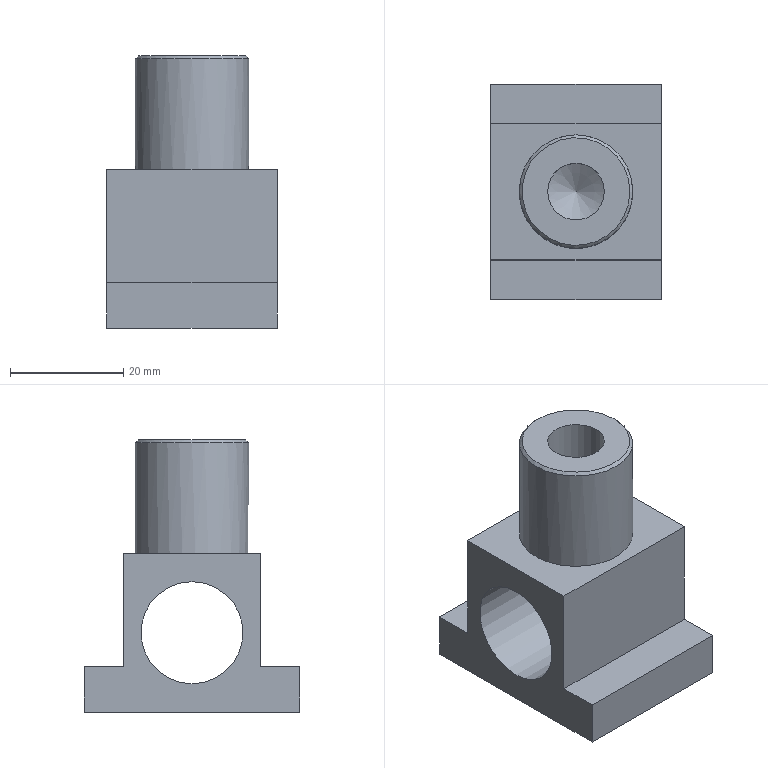Component | NX | 5 | 1 solid | 16 faces | box 30 x 38 x 48 mm | volume 20512 mm3 | plane 11 | cylinder 3 | cone 2 | commonest cylinder face diameters 18 x1 20 x1 10 x1
STEP:
#1=CARTESIAN_POINT('',(0.,0.,0.));
#2=DIRECTION('',(0.,0.,1.));
#3=DIRECTION('',(1.,0.,0.));
#4=AXIS2_PLACEMENT_3D('',#1,#2,#3);
#5=CARTESIAN_POINT('',(49.,-19.,9.));
#6=VERTEX_POINT('',#5);
#7=CARTESIAN_POINT('',(49.,-19.,1.));
#8=VERTEX_POINT('',#7);
#9=CARTESIAN_POINT('',(49.,-19.,9.));
#10=DIRECTION('',(0.,0.,-1.));
#11=VECTOR('',#10,1.);
#12=LINE('',#9,#11);
#13=CARTESIAN_POINT('',(79.,-19.,9.));
#14=DIRECTION('',(0.,1.,0.));
#15=DIRECTION('',(0.,0.,1.));
#16=AXIS2_PLACEMENT_3D('',#13,#14,#15);
#17=PLANE('',#16);
#18=CARTESIAN_POINT('',(0.,-30.));
#19=DIRECTION('',(-1.,0.));
#20=VECTOR('',#19,1.);
#21=LINE('',#18,#20);
#22=(GEOMETRIC_REPRESENTATION_CONTEXT(2)PARAMETRIC_REPRESENTATION_CONTEXT()REPRESENTATION_CONTEXT('',''));
#23=DEFINITIONAL_REPRESENTATION('',(#21),#22);
#24=PCURVE('',#17,#23);
#25=CARTESIAN_POINT('',(49.,-0.,1.));
#26=DIRECTION('',(1.,0.,0.));
#27=DIRECTION('',(0.,0.,-1.));
#28=AXIS2_PLACEMENT_3D('',#25,#26,#27);
#29=PLANE('',#28);
#30=CARTESIAN_POINT('',(-8.,-19.));
#31=DIRECTION('',(1.,0.));
#32=VECTOR('',#31,1.);
#33=LINE('',#30,#32);
#34=(GEOMETRIC_REPRESENTATION_CONTEXT(2)PARAMETRIC_REPRESENTATION_CONTEXT()REPRESENTATION_CONTEXT('',''));
#35=DEFINITIONAL_REPRESENTATION('',(#33),#34);
#36=PCURVE('',#29,#35);
#37=SURFACE_CURVE('',#12,(#24,#36),.PCURVE_S1.);
#38=EDGE_CURVE('',#6,#8,#37,.T.);
#39=ORIENTED_EDGE('',*,*,#38,.T.);
#40=CARTESIAN_POINT('',(79.,-19.,1.));
#41=VERTEX_POINT('',#40);
#42=CARTESIAN_POINT('',(79.,-19.,1.));
#43=DIRECTION('',(-1.,0.,0.));
#44=VECTOR('',#43,1.);
#45=LINE('',#42,#44);
#46=CARTESIAN_POINT('',(-8.,0.));
#47=DIRECTION('',(0.,-1.));
#48=VECTOR('',#47,1.);
#49=LINE('',#46,#48);
#50=(GEOMETRIC_REPRESENTATION_CONTEXT(2)PARAMETRIC_REPRESENTATION_CONTEXT()REPRESENTATION_CONTEXT('',''));
#51=DEFINITIONAL_REPRESENTATION('',(#49),#50);
#52=PCURVE('',#17,#51);
#53=CARTESIAN_POINT('',(79.,-19.,1.));
#54=DIRECTION('',(0.,-0.,1.));
#55=DIRECTION('',(0.,-1.,-0.));
#56=AXIS2_PLACEMENT_3D('',#53,#54,#55);
#57=PLANE('',#56);
#58=CARTESIAN_POINT('',(0.,0.));
#59=DIRECTION('',(0.,-1.));
#60=VECTOR('',#59,1.);
#61=LINE('',#58,#60);
#62=(GEOMETRIC_REPRESENTATION_CONTEXT(2)PARAMETRIC_REPRESENTATION_CONTEXT()REPRESENTATION_CONTEXT('',''));
#63=DEFINITIONAL_REPRESENTATION('',(#61),#62);
#64=PCURVE('',#57,#63);
#65=SURFACE_CURVE('',#45,(#52,#64),.PCURVE_S1.);
#66=EDGE_CURVE('',#41,#8,#65,.T.);
#67=ORIENTED_EDGE('',*,*,#66,.F.);
#68=CARTESIAN_POINT('',(79.,-19.,9.));
#69=VERTEX_POINT('',#68);
#70=CARTESIAN_POINT('',(79.,-19.,9.));
#71=DIRECTION('',(0.,0.,-1.));
#72=VECTOR('',#71,1.);
#73=LINE('',#70,#72);
#74=CARTESIAN_POINT('',(0.,0.));
#75=DIRECTION('',(-1.,0.));
#76=VECTOR('',#75,1.);
#77=LINE('',#74,#76);
#78=(GEOMETRIC_REPRESENTATION_CONTEXT(2)PARAMETRIC_REPRESENTATION_CONTEXT()REPRESENTATION_CONTEXT('',''));
#79=DEFINITIONAL_REPRESENTATION('',(#77),#78);
#80=PCURVE('',#17,#79);
#81=CARTESIAN_POINT('',(79.,-0.,1.));
#82=DIRECTION('',(1.,0.,0.));
#83=DIRECTION('',(0.,0.,-1.));
#84=AXIS2_PLACEMENT_3D('',#81,#82,#83);
#85=PLANE('',#84);
#86=CARTESIAN_POINT('',(-8.,-19.));
#87=DIRECTION('',(1.,0.));
#88=VECTOR('',#87,1.);
#89=LINE('',#86,#88);
#90=(GEOMETRIC_REPRESENTATION_CONTEXT(2)PARAMETRIC_REPRESENTATION_CONTEXT()REPRESENTATION_CONTEXT('',''));
#91=DEFINITIONAL_REPRESENTATION('',(#89),#90);
#92=PCURVE('',#85,#91);
#93=SURFACE_CURVE('',#73,(#80,#92),.PCURVE_S1.);
#94=EDGE_CURVE('',#69,#41,#93,.T.);
#95=ORIENTED_EDGE('',*,*,#94,.F.);
#96=CARTESIAN_POINT('',(79.,-19.,9.));
#97=DIRECTION('',(-1.,0.,0.));
#98=VECTOR('',#97,1.);
#99=LINE('',#96,#98);
#100=CARTESIAN_POINT('',(0.,0.));
#101=DIRECTION('',(0.,-1.));
#102=VECTOR('',#101,1.);
#103=LINE('',#100,#102);
#104=(GEOMETRIC_REPRESENTATION_CONTEXT(2)PARAMETRIC_REPRESENTATION_CONTEXT()REPRESENTATION_CONTEXT('',''));
#105=DEFINITIONAL_REPRESENTATION('',(#103),#104);
#106=PCURVE('',#17,#105);
#107=CARTESIAN_POINT('',(79.,-12.,9.));
#108=DIRECTION('',(0.,0.,-1.));
#109=DIRECTION('',(-1.,0.,0.));
#110=AXIS2_PLACEMENT_3D('',#107,#108,#109);
#111=PLANE('',#110);
#112=CARTESIAN_POINT('',(0.,-7.));
#113=DIRECTION('',(1.,0.));
#114=VECTOR('',#113,1.);
#115=LINE('',#112,#114);
#116=(GEOMETRIC_REPRESENTATION_CONTEXT(2)PARAMETRIC_REPRESENTATION_CONTEXT()REPRESENTATION_CONTEXT('',''));
#117=DEFINITIONAL_REPRESENTATION('',(#115),#116);
#118=PCURVE('',#111,#117);
#119=SURFACE_CURVE('',#99,(#106,#118),.PCURVE_S1.);
#120=EDGE_CURVE('',#69,#6,#119,.T.);
#121=ORIENTED_EDGE('',*,*,#120,.T.);
#122=EDGE_LOOP('',(#39,#67,#95,#121));
#123=FACE_BOUND('',#122,.T.);
#124=ADVANCED_FACE('',(#123),#17,.F.);
#125=CARTESIAN_POINT('',(49.,19.,1.));
#126=VERTEX_POINT('',#125);
#127=CARTESIAN_POINT('',(49.,-19.,1.));
#128=DIRECTION('',(0.,1.,0.));
#129=VECTOR('',#128,1.);
#130=LINE('',#127,#129);
#131=CARTESIAN_POINT('',(0.,-30.));
#132=DIRECTION('',(-1.,0.));
#133=VECTOR('',#132,1.);
#134=LINE('',#131,#133);
#135=(GEOMETRIC_REPRESENTATION_CONTEXT(2)PARAMETRIC_REPRESENTATION_CONTEXT()REPRESENTATION_CONTEXT('',''));
#136=DEFINITIONAL_REPRESENTATION('',(#134),#135);
#137=PCURVE('',#57,#136);
#138=CARTESIAN_POINT('',(0.,-19.));
#139=DIRECTION('',(-0.,1.));
#140=VECTOR('',#139,1.);
#141=LINE('',#138,#140);
#142=(GEOMETRIC_REPRESENTATION_CONTEXT(2)PARAMETRIC_REPRESENTATION_CONTEXT()REPRESENTATION_CONTEXT('',''));
#143=DEFINITIONAL_REPRESENTATION('',(#141),#142);
#144=PCURVE('',#29,#143);
#145=SURFACE_CURVE('',#130,(#137,#144),.PCURVE_S1.);
#146=EDGE_CURVE('',#8,#126,#145,.T.);
#147=ORIENTED_EDGE('',*,*,#146,.T.);
#148=CARTESIAN_POINT('',(79.,19.,1.));
#149=VERTEX_POINT('',#148);
#150=CARTESIAN_POINT('',(79.,19.,1.));
#151=DIRECTION('',(-1.,0.,0.));
#152=VECTOR('',#151,1.);
#153=LINE('',#150,#152);
#154=CARTESIAN_POINT('',(-38.,0.));
#155=DIRECTION('',(0.,-1.));
#156=VECTOR('',#155,1.);
#157=LINE('',#154,#156);
#158=(GEOMETRIC_REPRESENTATION_CONTEXT(2)PARAMETRIC_REPRESENTATION_CONTEXT()REPRESENTATION_CONTEXT('',''));
#159=DEFINITIONAL_REPRESENTATION('',(#157),#158);
#160=PCURVE('',#57,#159);
#161=CARTESIAN_POINT('',(79.,19.,1.));
#162=DIRECTION('',(0.,-1.,0.));
#163=DIRECTION('',(0.,0.,-1.));
#164=AXIS2_PLACEMENT_3D('',#161,#162,#163);
#165=PLANE('',#164);
#166=CARTESIAN_POINT('',(0.,0.));
#167=DIRECTION('',(0.,-1.));
#168=VECTOR('',#167,1.);
#169=LINE('',#166,#168);
#170=(GEOMETRIC_REPRESENTATION_CONTEXT(2)PARAMETRIC_REPRESENTATION_CONTEXT()REPRESENTATION_CONTEXT('',''));
#171=DEFINITIONAL_REPRESENTATION('',(#169),#170);
#172=PCURVE('',#165,#171);
#173=SURFACE_CURVE('',#153,(#160,#172),.PCURVE_S1.);
#174=EDGE_CURVE('',#149,#126,#173,.T.);
#175=ORIENTED_EDGE('',*,*,#174,.F.);
#176=CARTESIAN_POINT('',(79.,-19.,1.));
#177=DIRECTION('',(0.,1.,0.));
#178=VECTOR('',#177,1.);
#179=LINE('',#176,#178);
#180=CARTESIAN_POINT('',(0.,0.));
#181=DIRECTION('',(-1.,0.));
#182=VECTOR('',#181,1.);
#183=LINE('',#180,#182);
#184=(GEOMETRIC_REPRESENTATION_CONTEXT(2)PARAMETRIC_REPRESENTATION_CONTEXT()REPRESENTATION_CONTEXT('',''));
#185=DEFINITIONAL_REPRESENTATION('',(#183),#184);
#186=PCURVE('',#57,#185);
#187=CARTESIAN_POINT('',(0.,-19.));
#188=DIRECTION('',(-0.,1.));
#189=VECTOR('',#188,1.);
#190=LINE('',#187,#189);
#191=(GEOMETRIC_REPRESENTATION_CONTEXT(2)PARAMETRIC_REPRESENTATION_CONTEXT()REPRESENTATION_CONTEXT('',''));
#192=DEFINITIONAL_REPRESENTATION('',(#190),#191);
#193=PCURVE('',#85,#192);
#194=SURFACE_CURVE('',#179,(#186,#193),.PCURVE_S1.);
#195=EDGE_CURVE('',#41,#149,#194,.T.);
#196=ORIENTED_EDGE('',*,*,#195,.F.);
#197=ORIENTED_EDGE('',*,*,#66,.T.);
#198=EDGE_LOOP('',(#147,#175,#196,#197));
#199=FACE_BOUND('',#198,.T.);
#200=ADVANCED_FACE('',(#199),#57,.F.);
#201=CARTESIAN_POINT('',(49.,19.,9.));
#202=VERTEX_POINT('',#201);
#203=CARTESIAN_POINT('',(49.,19.,1.));
#204=DIRECTION('',(0.,0.,1.));
#205=VECTOR('',#204,1.);
#206=LINE('',#203,#205);
#207=CARTESIAN_POINT('',(0.,-30.));
#208=DIRECTION('',(-1.,0.));
#209=VECTOR('',#208,1.);
#210=LINE('',#207,#209);
#211=(GEOMETRIC_REPRESENTATION_CONTEXT(2)PARAMETRIC_REPRESENTATION_CONTEXT()REPRESENTATION_CONTEXT('',''));
#212=DEFINITIONAL_REPRESENTATION('',(#210),#211);
#213=PCURVE('',#165,#212);
#214=CARTESIAN_POINT('',(0.,19.));
#215=DIRECTION('',(-1.,0.));
#216=VECTOR('',#215,1.);
#217=LINE('',#214,#216);
#218=(GEOMETRIC_REPRESENTATION_CONTEXT(2)PARAMETRIC_REPRESENTATION_CONTEXT()REPRESENTATION_CONTEXT('',''));
#219=DEFINITIONAL_REPRESENTATION('',(#217),#218);
#220=PCURVE('',#29,#219);
#221=SURFACE_CURVE('',#206,(#213,#220),.PCURVE_S1.);
#222=EDGE_CURVE('',#126,#202,#221,.T.);
#223=ORIENTED_EDGE('',*,*,#222,.T.);
#224=CARTESIAN_POINT('',(79.,19.,9.));
#225=VERTEX_POINT('',#224);
#226=CARTESIAN_POINT('',(79.,19.,9.));
#227=DIRECTION('',(-1.,0.,0.));
#228=VECTOR('',#227,1.);
#229=LINE('',#226,#228);
#230=CARTESIAN_POINT('',(-8.,0.));
#231=DIRECTION('',(0.,-1.));
#232=VECTOR('',#231,1.);
#233=LINE('',#230,#232);
#234=(GEOMETRIC_REPRESENTATION_CONTEXT(2)PARAMETRIC_REPRESENTATION_CONTEXT()REPRESENTATION_CONTEXT('',''));
#235=DEFINITIONAL_REPRESENTATION('',(#233),#234);
#236=PCURVE('',#165,#235);
#237=CARTESIAN_POINT('',(79.,19.,9.));
#238=DIRECTION('',(0.,0.,-1.));
#239=DIRECTION('',(0.,1.,0.));
#240=AXIS2_PLACEMENT_3D('',#237,#238,#239);
#241=PLANE('',#240);
#242=CARTESIAN_POINT('',(0.,0.));
#243=DIRECTION('',(0.,-1.));
#244=VECTOR('',#243,1.);
#245=LINE('',#242,#244);
#246=(GEOMETRIC_REPRESENTATION_CONTEXT(2)PARAMETRIC_REPRESENTATION_CONTEXT()REPRESENTATION_CONTEXT('',''));
#247=DEFINITIONAL_REPRESENTATION('',(#245),#246);
#248=PCURVE('',#241,#247);
#249=SURFACE_CURVE('',#229,(#236,#248),.PCURVE_S1.);
#250=EDGE_CURVE('',#225,#202,#249,.T.);
#251=ORIENTED_EDGE('',*,*,#250,.F.);
#252=CARTESIAN_POINT('',(79.,19.,1.));
#253=DIRECTION('',(0.,0.,1.));
#254=VECTOR('',#253,1.);
#255=LINE('',#252,#254);
#256=CARTESIAN_POINT('',(0.,0.));
#257=DIRECTION('',(-1.,0.));
#258=VECTOR('',#257,1.);
#259=LINE('',#256,#258);
#260=(GEOMETRIC_REPRESENTATION_CONTEXT(2)PARAMETRIC_REPRESENTATION_CONTEXT()REPRESENTATION_CONTEXT('',''));
#261=DEFINITIONAL_REPRESENTATION('',(#259),#260);
#262=PCURVE('',#165,#261);
#263=CARTESIAN_POINT('',(0.,19.));
#264=DIRECTION('',(-1.,0.));
#265=VECTOR('',#264,1.);
#266=LINE('',#263,#265);
#267=(GEOMETRIC_REPRESENTATION_CONTEXT(2)PARAMETRIC_REPRESENTATION_CONTEXT()REPRESENTATION_CONTEXT('',''));
#268=DEFINITIONAL_REPRESENTATION('',(#266),#267);
#269=PCURVE('',#85,#268);
#270=SURFACE_CURVE('',#255,(#262,#269),.PCURVE_S1.);
#271=EDGE_CURVE('',#149,#225,#270,.T.);
#272=ORIENTED_EDGE('',*,*,#271,.F.);
#273=ORIENTED_EDGE('',*,*,#174,.T.);
#274=EDGE_LOOP('',(#223,#251,#272,#273));
#275=FACE_BOUND('',#274,.T.);
#276=ADVANCED_FACE('',(#275),#165,.F.);
#277=CARTESIAN_POINT('',(49.,12.,9.));
#278=VERTEX_POINT('',#277);
#279=CARTESIAN_POINT('',(49.,19.,9.));
#280=DIRECTION('',(0.,-1.,-0.));
#281=VECTOR('',#280,1.);
#282=LINE('',#279,#281);
#283=CARTESIAN_POINT('',(0.,-30.));
#284=DIRECTION('',(-1.,0.));
#285=VECTOR('',#284,1.);
#286=LINE('',#283,#285);
#287=(GEOMETRIC_REPRESENTATION_CONTEXT(2)PARAMETRIC_REPRESENTATION_CONTEXT()REPRESENTATION_CONTEXT('',''));
#288=DEFINITIONAL_REPRESENTATION('',(#286),#287);
#289=PCURVE('',#241,#288);
#290=CARTESIAN_POINT('',(-8.,19.));
#291=DIRECTION('',(0.,-1.));
#292=VECTOR('',#291,1.);
#293=LINE('',#290,#292);
#294=(GEOMETRIC_REPRESENTATION_CONTEXT(2)PARAMETRIC_REPRESENTATION_CONTEXT()REPRESENTATION_CONTEXT('',''));
#295=DEFINITIONAL_REPRESENTATION('',(#293),#294);
#296=PCURVE('',#29,#295);
#297=SURFACE_CURVE('',#282,(#289,#296),.PCURVE_S1.);
#298=EDGE_CURVE('',#202,#278,#297,.T.);
#299=ORIENTED_EDGE('',*,*,#298,.T.);
#300=CARTESIAN_POINT('',(79.,12.,9.));
#301=VERTEX_POINT('',#300);
#302=CARTESIAN_POINT('',(79.,12.,9.));
#303=DIRECTION('',(-1.,0.,0.));
#304=VECTOR('',#303,1.);
#305=LINE('',#302,#304);
#306=CARTESIAN_POINT('',(-7.,0.));
#307=DIRECTION('',(0.,-1.));
#308=VECTOR('',#307,1.);
#309=LINE('',#306,#308);
#310=(GEOMETRIC_REPRESENTATION_CONTEXT(2)PARAMETRIC_REPRESENTATION_CONTEXT()REPRESENTATION_CONTEXT('',''));
#311=DEFINITIONAL_REPRESENTATION('',(#309),#310);
#312=PCURVE('',#241,#311);
#313=CARTESIAN_POINT('',(79.,12.,9.));
#314=DIRECTION('',(0.,-1.,-0.));
#315=DIRECTION('',(0.,0.,-1.));
#316=AXIS2_PLACEMENT_3D('',#313,#314,#315);
#317=PLANE('',#316);
#318=CARTESIAN_POINT('',(0.,0.));
#319=DIRECTION('',(0.,-1.));
#320=VECTOR('',#319,1.);
#321=LINE('',#318,#320);
#322=(GEOMETRIC_REPRESENTATION_CONTEXT(2)PARAMETRIC_REPRESENTATION_CONTEXT()REPRESENTATION_CONTEXT('',''));
#323=DEFINITIONAL_REPRESENTATION('',(#321),#322);
#324=PCURVE('',#317,#323);
#325=SURFACE_CURVE('',#305,(#312,#324),.PCURVE_S1.);
#326=EDGE_CURVE('',#301,#278,#325,.T.);
#327=ORIENTED_EDGE('',*,*,#326,.F.);
#328=CARTESIAN_POINT('',(79.,19.,9.));
#329=DIRECTION('',(0.,-1.,-0.));
#330=VECTOR('',#329,1.);
#331=LINE('',#328,#330);
#332=CARTESIAN_POINT('',(0.,0.));
#333=DIRECTION('',(-1.,0.));
#334=VECTOR('',#333,1.);
#335=LINE('',#332,#334);
#336=(GEOMETRIC_REPRESENTATION_CONTEXT(2)PARAMETRIC_REPRESENTATION_CONTEXT()REPRESENTATION_CONTEXT('',''));
#337=DEFINITIONAL_REPRESENTATION('',(#335),#336);
#338=PCURVE('',#241,#337);
#339=CARTESIAN_POINT('',(-8.,19.));
#340=DIRECTION('',(0.,-1.));
#341=VECTOR('',#340,1.);
#342=LINE('',#339,#341);
#343=(GEOMETRIC_REPRESENTATION_CONTEXT(2)PARAMETRIC_REPRESENTATION_CONTEXT()REPRESENTATION_CONTEXT('',''));
#344=DEFINITIONAL_REPRESENTATION('',(#342),#343);
#345=PCURVE('',#85,#344);
#346=SURFACE_CURVE('',#331,(#338,#345),.PCURVE_S1.);
#347=EDGE_CURVE('',#225,#301,#346,.T.);
#348=ORIENTED_EDGE('',*,*,#347,.F.);
#349=ORIENTED_EDGE('',*,*,#250,.T.);
#350=EDGE_LOOP('',(#299,#327,#348,#349));
#351=FACE_BOUND('',#350,.T.);
#352=ADVANCED_FACE('',(#351),#241,.F.);
#353=CARTESIAN_POINT('',(49.,12.,29.));
#354=VERTEX_POINT('',#353);
#355=CARTESIAN_POINT('',(49.,12.,9.));
#356=DIRECTION('',(0.,-0.,1.));
#357=VECTOR('',#356,1.);
#358=LINE('',#355,#357);
#359=CARTESIAN_POINT('',(0.,-30.));
#360=DIRECTION('',(-1.,0.));
#361=VECTOR('',#360,1.);
#362=LINE('',#359,#361);
#363=(GEOMETRIC_REPRESENTATION_CONTEXT(2)PARAMETRIC_REPRESENTATION_CONTEXT()REPRESENTATION_CONTEXT('',''));
#364=DEFINITIONAL_REPRESENTATION('',(#362),#363);
#365=PCURVE('',#317,#364);
#366=CARTESIAN_POINT('',(-8.,12.));
#367=DIRECTION('',(-1.,-0.));
#368=VECTOR('',#367,1.);
#369=LINE('',#366,#368);
#370=(GEOMETRIC_REPRESENTATION_CONTEXT(2)PARAMETRIC_REPRESENTATION_CONTEXT()REPRESENTATION_CONTEXT('',''));
#371=DEFINITIONAL_REPRESENTATION('',(#369),#370);
#372=PCURVE('',#29,#371);
#373=SURFACE_CURVE('',#358,(#365,#372),.PCURVE_S1.);
#374=EDGE_CURVE('',#278,#354,#373,.T.);
#375=ORIENTED_EDGE('',*,*,#374,.T.);
#376=CARTESIAN_POINT('',(79.,12.,29.));
#377=VERTEX_POINT('',#376);
#378=CARTESIAN_POINT('',(79.,12.,29.));
#379=DIRECTION('',(-1.,0.,0.));
#380=VECTOR('',#379,1.);
#381=LINE('',#378,#380);
#382=CARTESIAN_POINT('',(-20.,0.));
#383=DIRECTION('',(0.,-1.));
#384=VECTOR('',#383,1.);
#385=LINE('',#382,#384);
#386=(GEOMETRIC_REPRESENTATION_CONTEXT(2)PARAMETRIC_REPRESENTATION_CONTEXT()REPRESENTATION_CONTEXT('',''));
#387=DEFINITIONAL_REPRESENTATION('',(#385),#386);
#388=PCURVE('',#317,#387);
#389=CARTESIAN_POINT('',(79.,12.,29.));
#390=DIRECTION('',(0.,0.,-1.));
#391=DIRECTION('',(-1.,0.,0.));
#392=AXIS2_PLACEMENT_3D('',#389,#390,#391);
#393=PLANE('',#392);
#394=CARTESIAN_POINT('',(0.,0.));
#395=DIRECTION('',(1.,0.));
#396=VECTOR('',#395,1.);
#397=LINE('',#394,#396);
#398=(GEOMETRIC_REPRESENTATION_CONTEXT(2)PARAMETRIC_REPRESENTATION_CONTEXT()REPRESENTATION_CONTEXT('',''));
#399=DEFINITIONAL_REPRESENTATION('',(#397),#398);
#400=PCURVE('',#393,#399);
#401=SURFACE_CURVE('',#381,(#388,#400),.PCURVE_S1.);
#402=EDGE_CURVE('',#377,#354,#401,.T.);
#403=ORIENTED_EDGE('',*,*,#402,.F.);
#404=CARTESIAN_POINT('',(79.,12.,9.));
#405=DIRECTION('',(0.,-0.,1.));
#406=VECTOR('',#405,1.);
#407=LINE('',#404,#406);
#408=CARTESIAN_POINT('',(0.,0.));
#409=DIRECTION('',(-1.,0.));
#410=VECTOR('',#409,1.);
#411=LINE('',#408,#410);
#412=(GEOMETRIC_REPRESENTATION_CONTEXT(2)PARAMETRIC_REPRESENTATION_CONTEXT()REPRESENTATION_CONTEXT('',''));
#413=DEFINITIONAL_REPRESENTATION('',(#411),#412);
#414=PCURVE('',#317,#413);
#415=CARTESIAN_POINT('',(-8.,12.));
#416=DIRECTION('',(-1.,-0.));
#417=VECTOR('',#416,1.);
#418=LINE('',#415,#417);
#419=(GEOMETRIC_REPRESENTATION_CONTEXT(2)PARAMETRIC_REPRESENTATION_CONTEXT()REPRESENTATION_CONTEXT('',''));
#420=DEFINITIONAL_REPRESENTATION('',(#418),#419);
#421=PCURVE('',#85,#420);
#422=SURFACE_CURVE('',#407,(#414,#421),.PCURVE_S1.);
#423=EDGE_CURVE('',#301,#377,#422,.T.);
#424=ORIENTED_EDGE('',*,*,#423,.F.);
#425=ORIENTED_EDGE('',*,*,#326,.T.);
#426=EDGE_LOOP('',(#375,#403,#424,#425));
#427=FACE_BOUND('',#426,.T.);
#428=ADVANCED_FACE('',(#427),#317,.F.);
#429=CARTESIAN_POINT('',(64.,10.,29.));
#430=VERTEX_POINT('',#429);
#431=CARTESIAN_POINT('',(64.,-0.,29.));
#432=DIRECTION('',(0.,0.,1.));
#433=DIRECTION('',(0.,1.,0.));
#434=AXIS2_PLACEMENT_3D('',#431,#432,#433);
#435=CIRCLE('',#434,10.);
#436=CARTESIAN_POINT('',(15.,-2.));
#437=CARTESIAN_POINT('',(32.321,-2.));
#438=CARTESIAN_POINT('',(23.66,-17.));
#439=CARTESIAN_POINT('',(15.,-32.));
#440=CARTESIAN_POINT('',(6.34,-17.));
#441=CARTESIAN_POINT('',(-2.321,-2.));
#442=CARTESIAN_POINT('',(15.,-2.));
#443=(BOUNDED_CURVE()B_SPLINE_CURVE(2,(#436,#437,#438,#439,#440,#441,#442),.UNSPECIFIED.,.T.,.F.)B_SPLINE_CURVE_WITH_KNOTS((1,2,2,2,2,1),(-2.094,0.,2.094,4.189,6.283,8.378),.UNSPECIFIED.)CURVE()GEOMETRIC_REPRESENTATION_ITEM()RATIONAL_B_SPLINE_CURVE((1.,0.5,1.,0.5,1.,0.5,1.))REPRESENTATION_ITEM(''));
#444=(GEOMETRIC_REPRESENTATION_CONTEXT(2)PARAMETRIC_REPRESENTATION_CONTEXT()REPRESENTATION_CONTEXT('',''));
#445=DEFINITIONAL_REPRESENTATION('',(#443),#444);
#446=PCURVE('',#393,#445);
#447=CARTESIAN_POINT('',(64.,-0.,49.));
#448=DIRECTION('',(0.,0.,-1.));
#449=DIRECTION('',(-1.,0.,0.));
#450=AXIS2_PLACEMENT_3D('',#447,#448,#449);
#451=CYLINDRICAL_SURFACE('',#450,10.);
#452=CARTESIAN_POINT('',(7.854,20.));
#453=DIRECTION('',(-1.,0.));
#454=VECTOR('',#453,1.);
#455=LINE('',#452,#454);
#456=(GEOMETRIC_REPRESENTATION_CONTEXT(2)PARAMETRIC_REPRESENTATION_CONTEXT()REPRESENTATION_CONTEXT('',''));
#457=DEFINITIONAL_REPRESENTATION('',(#455),#456);
#458=PCURVE('',#451,#457);
#459=SURFACE_CURVE('',#435,(#446,#458),.PCURVE_S1.);
#460=EDGE_CURVE('',#430,#430,#459,.T.);
#461=ORIENTED_EDGE('',*,*,#460,.F.);
#462=EDGE_LOOP('',(#461));
#463=FACE_BOUND('',#462,.T.);
#464=CARTESIAN_POINT('',(49.,-12.,29.));
#465=VERTEX_POINT('',#464);
#466=CARTESIAN_POINT('',(49.,12.,29.));
#467=DIRECTION('',(0.,-1.,0.));
#468=VECTOR('',#467,1.);
#469=LINE('',#466,#468);
#470=CARTESIAN_POINT('',(30.,0.));
#471=DIRECTION('',(0.,-1.));
#472=VECTOR('',#471,1.);
#473=LINE('',#470,#472);
#474=(GEOMETRIC_REPRESENTATION_CONTEXT(2)PARAMETRIC_REPRESENTATION_CONTEXT()REPRESENTATION_CONTEXT('',''));
#475=DEFINITIONAL_REPRESENTATION('',(#473),#474);
#476=PCURVE('',#393,#475);
#477=CARTESIAN_POINT('',(-28.,12.));
#478=DIRECTION('',(0.,-1.));
#479=VECTOR('',#478,1.);
#480=LINE('',#477,#479);
#481=(GEOMETRIC_REPRESENTATION_CONTEXT(2)PARAMETRIC_REPRESENTATION_CONTEXT()REPRESENTATION_CONTEXT('',''));
#482=DEFINITIONAL_REPRESENTATION('',(#480),#481);
#483=PCURVE('',#29,#482);
#484=SURFACE_CURVE('',#469,(#476,#483),.PCURVE_S1.);
#485=EDGE_CURVE('',#354,#465,#484,.T.);
#486=ORIENTED_EDGE('',*,*,#485,.T.);
#487=CARTESIAN_POINT('',(79.,-12.,29.));
#488=VERTEX_POINT('',#487);
#489=CARTESIAN_POINT('',(79.,-12.,29.));
#490=DIRECTION('',(-1.,0.,0.));
#491=VECTOR('',#490,1.);
#492=LINE('',#489,#491);
#493=CARTESIAN_POINT('',(0.,-24.));
#494=DIRECTION('',(1.,0.));
#495=VECTOR('',#494,1.);
#496=LINE('',#493,#495);
#497=(GEOMETRIC_REPRESENTATION_CONTEXT(2)PARAMETRIC_REPRESENTATION_CONTEXT()REPRESENTATION_CONTEXT('',''));
#498=DEFINITIONAL_REPRESENTATION('',(#496),#497);
#499=PCURVE('',#393,#498);
#500=CARTESIAN_POINT('',(79.,-12.,29.));
#501=DIRECTION('',(0.,1.,-0.));
#502=DIRECTION('',(0.,0.,1.));
#503=AXIS2_PLACEMENT_3D('',#500,#501,#502);
#504=PLANE('',#503);
#505=CARTESIAN_POINT('',(0.,0.));
#506=DIRECTION('',(0.,-1.));
#507=VECTOR('',#506,1.);
#508=LINE('',#505,#507);
#509=(GEOMETRIC_REPRESENTATION_CONTEXT(2)PARAMETRIC_REPRESENTATION_CONTEXT()REPRESENTATION_CONTEXT('',''));
#510=DEFINITIONAL_REPRESENTATION('',(#508),#509);
#511=PCURVE('',#504,#510);
#512=SURFACE_CURVE('',#492,(#499,#511),.PCURVE_S1.);
#513=EDGE_CURVE('',#488,#465,#512,.T.);
#514=ORIENTED_EDGE('',*,*,#513,.F.);
#515=CARTESIAN_POINT('',(79.,12.,29.));
#516=DIRECTION('',(0.,-1.,0.));
#517=VECTOR('',#516,1.);
#518=LINE('',#515,#517);
#519=CARTESIAN_POINT('',(0.,0.));
#520=DIRECTION('',(0.,-1.));
#521=VECTOR('',#520,1.);
#522=LINE('',#519,#521);
#523=(GEOMETRIC_REPRESENTATION_CONTEXT(2)PARAMETRIC_REPRESENTATION_CONTEXT()REPRESENTATION_CONTEXT('',''));
#524=DEFINITIONAL_REPRESENTATION('',(#522),#523);
#525=PCURVE('',#393,#524);
#526=CARTESIAN_POINT('',(-28.,12.));
#527=DIRECTION('',(0.,-1.));
#528=VECTOR('',#527,1.);
#529=LINE('',#526,#528);
#530=(GEOMETRIC_REPRESENTATION_CONTEXT(2)PARAMETRIC_REPRESENTATION_CONTEXT()REPRESENTATION_CONTEXT('',''));
#531=DEFINITIONAL_REPRESENTATION('',(#529),#530);
#532=PCURVE('',#85,#531);
#533=SURFACE_CURVE('',#518,(#525,#532),.PCURVE_S1.);
#534=EDGE_CURVE('',#377,#488,#533,.T.);
#535=ORIENTED_EDGE('',*,*,#534,.F.);
#536=ORIENTED_EDGE('',*,*,#402,.T.);
#537=EDGE_LOOP('',(#486,#514,#535,#536));
#538=FACE_BOUND('',#537,.T.);
#539=ADVANCED_FACE('',(#463,#538),#393,.F.);
#540=CARTESIAN_POINT('',(49.,-12.,9.));
#541=VERTEX_POINT('',#540);
#542=CARTESIAN_POINT('',(49.,-12.,29.));
#543=DIRECTION('',(0.,-0.,-1.));
#544=VECTOR('',#543,1.);
#545=LINE('',#542,#544);
#546=CARTESIAN_POINT('',(0.,-30.));
#547=DIRECTION('',(-1.,0.));
#548=VECTOR('',#547,1.);
#549=LINE('',#546,#548);
#550=(GEOMETRIC_REPRESENTATION_CONTEXT(2)PARAMETRIC_REPRESENTATION_CONTEXT()REPRESENTATION_CONTEXT('',''));
#551=DEFINITIONAL_REPRESENTATION('',(#549),#550);
#552=PCURVE('',#504,#551);
#553=CARTESIAN_POINT('',(-28.,-12.));
#554=DIRECTION('',(1.,-0.));
#555=VECTOR('',#554,1.);
#556=LINE('',#553,#555);
#557=(GEOMETRIC_REPRESENTATION_CONTEXT(2)PARAMETRIC_REPRESENTATION_CONTEXT()REPRESENTATION_CONTEXT('',''));
#558=DEFINITIONAL_REPRESENTATION('',(#556),#557);
#559=PCURVE('',#29,#558);
#560=SURFACE_CURVE('',#545,(#552,#559),.PCURVE_S1.);
#561=EDGE_CURVE('',#465,#541,#560,.T.);
#562=ORIENTED_EDGE('',*,*,#561,.T.);
#563=CARTESIAN_POINT('',(79.,-12.,9.));
#564=VERTEX_POINT('',#563);
#565=CARTESIAN_POINT('',(79.,-12.,9.));
#566=DIRECTION('',(-1.,0.,0.));
#567=VECTOR('',#566,1.);
#568=LINE('',#565,#567);
#569=CARTESIAN_POINT('',(-20.,0.));
#570=DIRECTION('',(0.,-1.));
#571=VECTOR('',#570,1.);
#572=LINE('',#569,#571);
#573=(GEOMETRIC_REPRESENTATION_CONTEXT(2)PARAMETRIC_REPRESENTATION_CONTEXT()REPRESENTATION_CONTEXT('',''));
#574=DEFINITIONAL_REPRESENTATION('',(#572),#573);
#575=PCURVE('',#504,#574);
#576=CARTESIAN_POINT('',(0.,0.));
#577=DIRECTION('',(1.,0.));
#578=VECTOR('',#577,1.);
#579=LINE('',#576,#578);
#580=(GEOMETRIC_REPRESENTATION_CONTEXT(2)PARAMETRIC_REPRESENTATION_CONTEXT()REPRESENTATION_CONTEXT('',''));
#581=DEFINITIONAL_REPRESENTATION('',(#579),#580);
#582=PCURVE('',#111,#581);
#583=SURFACE_CURVE('',#568,(#575,#582),.PCURVE_S1.);
#584=EDGE_CURVE('',#564,#541,#583,.T.);
#585=ORIENTED_EDGE('',*,*,#584,.F.);
#586=CARTESIAN_POINT('',(79.,-12.,29.));
#587=DIRECTION('',(0.,-0.,-1.));
#588=VECTOR('',#587,1.);
#589=LINE('',#586,#588);
#590=CARTESIAN_POINT('',(0.,0.));
#591=DIRECTION('',(-1.,0.));
#592=VECTOR('',#591,1.);
#593=LINE('',#590,#592);
#594=(GEOMETRIC_REPRESENTATION_CONTEXT(2)PARAMETRIC_REPRESENTATION_CONTEXT()REPRESENTATION_CONTEXT('',''));
#595=DEFINITIONAL_REPRESENTATION('',(#593),#594);
#596=PCURVE('',#504,#595);
#597=CARTESIAN_POINT('',(-28.,-12.));
#598=DIRECTION('',(1.,-0.));
#599=VECTOR('',#598,1.);
#600=LINE('',#597,#599);
#601=(GEOMETRIC_REPRESENTATION_CONTEXT(2)PARAMETRIC_REPRESENTATION_CONTEXT()REPRESENTATION_CONTEXT('',''));
#602=DEFINITIONAL_REPRESENTATION('',(#600),#601);
#603=PCURVE('',#85,#602);
#604=SURFACE_CURVE('',#589,(#596,#603),.PCURVE_S1.);
#605=EDGE_CURVE('',#488,#564,#604,.T.);
#606=ORIENTED_EDGE('',*,*,#605,.F.);
#607=ORIENTED_EDGE('',*,*,#513,.T.);
#608=EDGE_LOOP('',(#562,#585,#606,#607));
#609=FACE_BOUND('',#608,.T.);
#610=ADVANCED_FACE('',(#609),#504,.F.);
#611=CARTESIAN_POINT('',(49.,-12.,9.));
#612=DIRECTION('',(0.,-1.,0.));
#613=VECTOR('',#612,1.);
#614=LINE('',#611,#613);
#615=CARTESIAN_POINT('',(30.,0.));
#616=DIRECTION('',(0.,-1.));
#617=VECTOR('',#616,1.);
#618=LINE('',#615,#617);
#619=(GEOMETRIC_REPRESENTATION_CONTEXT(2)PARAMETRIC_REPRESENTATION_CONTEXT()REPRESENTATION_CONTEXT('',''));
#620=DEFINITIONAL_REPRESENTATION('',(#618),#619);
#621=PCURVE('',#111,#620);
#622=CARTESIAN_POINT('',(-8.,-12.));
#623=DIRECTION('',(0.,-1.));
#624=VECTOR('',#623,1.);
#625=LINE('',#622,#624);
#626=(GEOMETRIC_REPRESENTATION_CONTEXT(2)PARAMETRIC_REPRESENTATION_CONTEXT()REPRESENTATION_CONTEXT('',''));
#627=DEFINITIONAL_REPRESENTATION('',(#625),#626);
#628=PCURVE('',#29,#627);
#629=SURFACE_CURVE('',#614,(#621,#628),.PCURVE_S1.);
#630=EDGE_CURVE('',#541,#6,#629,.T.);
#631=ORIENTED_EDGE('',*,*,#630,.T.);
#632=ORIENTED_EDGE('',*,*,#120,.F.);
#633=CARTESIAN_POINT('',(79.,-12.,9.));
#634=DIRECTION('',(0.,-1.,0.));
#635=VECTOR('',#634,1.);
#636=LINE('',#633,#635);
#637=CARTESIAN_POINT('',(0.,0.));
#638=DIRECTION('',(0.,-1.));
#639=VECTOR('',#638,1.);
#640=LINE('',#637,#639);
#641=(GEOMETRIC_REPRESENTATION_CONTEXT(2)PARAMETRIC_REPRESENTATION_CONTEXT()REPRESENTATION_CONTEXT('',''));
#642=DEFINITIONAL_REPRESENTATION('',(#640),#641);
#643=PCURVE('',#111,#642);
#644=CARTESIAN_POINT('',(-8.,-12.));
#645=DIRECTION('',(0.,-1.));
#646=VECTOR('',#645,1.);
#647=LINE('',#644,#646);
#648=(GEOMETRIC_REPRESENTATION_CONTEXT(2)PARAMETRIC_REPRESENTATION_CONTEXT()REPRESENTATION_CONTEXT('',''));
#649=DEFINITIONAL_REPRESENTATION('',(#647),#648);
#650=PCURVE('',#85,#649);
#651=SURFACE_CURVE('',#636,(#643,#650),.PCURVE_S1.);
#652=EDGE_CURVE('',#564,#69,#651,.T.);
#653=ORIENTED_EDGE('',*,*,#652,.F.);
#654=ORIENTED_EDGE('',*,*,#584,.T.);
#655=EDGE_LOOP('',(#631,#632,#653,#654));
#656=FACE_BOUND('',#655,.T.);
#657=ADVANCED_FACE('',(#656),#111,.F.);
#658=CARTESIAN_POINT('',(79.,-0.,6.));
#659=VERTEX_POINT('',#658);
#660=CARTESIAN_POINT('',(79.,-0.,15.));
#661=DIRECTION('',(1.,0.,0.));
#662=DIRECTION('',(0.,0.,-1.));
#663=AXIS2_PLACEMENT_3D('',#660,#661,#662);
#664=CIRCLE('',#663,9.);
#665=CARTESIAN_POINT('',(-14.,0.));
#666=DIRECTION('',(1.,0.));
#667=AXIS2_PLACEMENT_2D('',#665,#666);
#668=CIRCLE('',#667,9.);
#669=(GEOMETRIC_REPRESENTATION_CONTEXT(2)PARAMETRIC_REPRESENTATION_CONTEXT()REPRESENTATION_CONTEXT('',''));
#670=DEFINITIONAL_REPRESENTATION('',(#668),#669);
#671=PCURVE('',#85,#670);
#672=CARTESIAN_POINT('',(6.,-0.,15.));
#673=DIRECTION('',(1.,0.,0.));
#674=DIRECTION('',(0.,0.,-1.));
#675=AXIS2_PLACEMENT_3D('',#672,#673,#674);
#676=CYLINDRICAL_SURFACE('',#675,9.);
#677=CARTESIAN_POINT('',(0.,73.));
#678=DIRECTION('',(1.,0.));
#679=VECTOR('',#678,1.);
#680=LINE('',#677,#679);
#681=(GEOMETRIC_REPRESENTATION_CONTEXT(2)PARAMETRIC_REPRESENTATION_CONTEXT()REPRESENTATION_CONTEXT('',''));
#682=DEFINITIONAL_REPRESENTATION('',(#680),#681);
#683=PCURVE('',#676,#682);
#684=SURFACE_CURVE('',#664,(#671,#683),.PCURVE_S1.);
#685=EDGE_CURVE('',#659,#659,#684,.T.);
#686=ORIENTED_EDGE('',*,*,#685,.F.);
#687=EDGE_LOOP('',(#686));
#688=FACE_BOUND('',#687,.T.);
#689=ORIENTED_EDGE('',*,*,#94,.T.);
#690=ORIENTED_EDGE('',*,*,#195,.T.);
#691=ORIENTED_EDGE('',*,*,#271,.T.);
#692=ORIENTED_EDGE('',*,*,#347,.T.);
#693=ORIENTED_EDGE('',*,*,#423,.T.);
#694=ORIENTED_EDGE('',*,*,#534,.T.);
#695=ORIENTED_EDGE('',*,*,#605,.T.);
#696=ORIENTED_EDGE('',*,*,#652,.T.);
#697=EDGE_LOOP('',(#689,#690,#691,#692,#693,#694,#695,#696));
#698=FACE_BOUND('',#697,.T.);
#699=ADVANCED_FACE('',(#688,#698),#85,.T.);
#700=CARTESIAN_POINT('',(49.,-0.,6.));
#701=VERTEX_POINT('',#700);
#702=CARTESIAN_POINT('',(49.,-0.,15.));
#703=DIRECTION('',(1.,0.,0.));
#704=DIRECTION('',(0.,0.,-1.));
#705=AXIS2_PLACEMENT_3D('',#702,#703,#704);
#706=CIRCLE('',#705,9.);
#707=CARTESIAN_POINT('',(-14.,0.));
#708=DIRECTION('',(1.,0.));
#709=AXIS2_PLACEMENT_2D('',#707,#708);
#710=CIRCLE('',#709,9.);
#711=(GEOMETRIC_REPRESENTATION_CONTEXT(2)PARAMETRIC_REPRESENTATION_CONTEXT()REPRESENTATION_CONTEXT('',''));
#712=DEFINITIONAL_REPRESENTATION('',(#710),#711);
#713=PCURVE('',#29,#712);
#714=CARTESIAN_POINT('',(0.,43.));
#715=DIRECTION('',(1.,0.));
#716=VECTOR('',#715,1.);
#717=LINE('',#714,#716);
#718=(GEOMETRIC_REPRESENTATION_CONTEXT(2)PARAMETRIC_REPRESENTATION_CONTEXT()REPRESENTATION_CONTEXT('',''));
#719=DEFINITIONAL_REPRESENTATION('',(#717),#718);
#720=PCURVE('',#676,#719);
#721=SURFACE_CURVE('',#706,(#713,#720),.PCURVE_S1.);
#722=EDGE_CURVE('',#701,#701,#721,.T.);
#723=ORIENTED_EDGE('',*,*,#722,.T.);
#724=EDGE_LOOP('',(#723));
#725=FACE_BOUND('',#724,.T.);
#726=ORIENTED_EDGE('',*,*,#38,.F.);
#727=ORIENTED_EDGE('',*,*,#630,.F.);
#728=ORIENTED_EDGE('',*,*,#561,.F.);
#729=ORIENTED_EDGE('',*,*,#485,.F.);
#730=ORIENTED_EDGE('',*,*,#374,.F.);
#731=ORIENTED_EDGE('',*,*,#298,.F.);
#732=ORIENTED_EDGE('',*,*,#222,.F.);
#733=ORIENTED_EDGE('',*,*,#146,.F.);
#734=EDGE_LOOP('',(#726,#727,#728,#729,#730,#731,#732,#733));
#735=FACE_BOUND('',#734,.T.);
#736=ADVANCED_FACE('',(#725,#735),#29,.F.);
#737=ORIENTED_EDGE('',*,*,#685,.F.);
#738=CARTESIAN_POINT('',(49.,-0.,6.));
#739=CARTESIAN_POINT('',(79.,-0.,6.));
#740=B_SPLINE_CURVE_WITH_KNOTS('',1,(#738,#739),.UNSPECIFIED.,.F.,.F.,(2,2),(43.,73.),.PIECEWISE_BEZIER_KNOTS.);
#741=CARTESIAN_POINT('',(0.,0.));
#742=DIRECTION('',(0.,1.));
#743=VECTOR('',#742,1.);
#744=LINE('',#741,#743);
#745=(GEOMETRIC_REPRESENTATION_CONTEXT(2)PARAMETRIC_REPRESENTATION_CONTEXT()REPRESENTATION_CONTEXT('',''));
#746=DEFINITIONAL_REPRESENTATION('',(#744),#745);
#747=PCURVE('',#676,#746);
#748=CARTESIAN_POINT('',(6.283,0.));
#749=DIRECTION('',(0.,1.));
#750=VECTOR('',#749,1.);
#751=LINE('',#748,#750);
#752=(GEOMETRIC_REPRESENTATION_CONTEXT(2)PARAMETRIC_REPRESENTATION_CONTEXT()REPRESENTATION_CONTEXT('',''));
#753=DEFINITIONAL_REPRESENTATION('',(#751),#752);
#754=PCURVE('',#676,#753);
#755=SEAM_CURVE('',#740,(#747,#754),.PCURVE_S1.);
#756=EDGE_CURVE('',#701,#659,#755,.T.);
#757=ORIENTED_EDGE('',*,*,#756,.F.);
#758=ORIENTED_EDGE('',*,*,#722,.T.);
#759=ORIENTED_EDGE('',*,*,#756,.T.);
#760=EDGE_LOOP('',(#737,#757,#758,#759));
#761=FACE_BOUND('',#760,.F.);
#762=ADVANCED_FACE('',(#761),#676,.F.);
#763=CARTESIAN_POINT('',(74.,-0.,48.5));
#764=VERTEX_POINT('',#763);
#765=CARTESIAN_POINT('',(64.,10.,48.5));
#766=VERTEX_POINT('',#765);
#767=CARTESIAN_POINT('',(64.,-0.,48.5));
#768=DIRECTION('',(0.,0.,-1.));
#769=DIRECTION('',(1.,0.,0.));
#770=AXIS2_PLACEMENT_3D('',#767,#768,#769);
#771=CIRCLE('',#770,10.);
#772=CARTESIAN_POINT('',(3.142,0.5));
#773=DIRECTION('',(1.,0.));
#774=VECTOR('',#773,1.);
#775=LINE('',#772,#774);
#776=(GEOMETRIC_REPRESENTATION_CONTEXT(2)PARAMETRIC_REPRESENTATION_CONTEXT()REPRESENTATION_CONTEXT('',''));
#777=DEFINITIONAL_REPRESENTATION('',(#775),#776);
#778=PCURVE('',#451,#777);
#779=CARTESIAN_POINT('',(64.,-0.,49.));
#780=DIRECTION('',(0.,0.,-1.));
#781=DIRECTION('',(-1.,0.,0.));
#782=AXIS2_PLACEMENT_3D('',#779,#780,#781);
#783=CONICAL_SURFACE('',#782,9.5,0.7854);
#784=CARTESIAN_POINT('',(3.142,0.5));
#785=DIRECTION('',(1.,0.));
#786=VECTOR('',#785,1.);
#787=LINE('',#784,#786);
#788=(GEOMETRIC_REPRESENTATION_CONTEXT(2)PARAMETRIC_REPRESENTATION_CONTEXT()REPRESENTATION_CONTEXT('',''));
#789=DEFINITIONAL_REPRESENTATION('',(#787),#788);
#790=PCURVE('',#783,#789);
#791=SURFACE_CURVE('',#771,(#778,#790),.PCURVE_S1.);
#792=EDGE_CURVE('',#764,#766,#791,.T.);
#793=ORIENTED_EDGE('',*,*,#792,.T.);
#794=CARTESIAN_POINT('',(64.,10.,48.5));
#795=CARTESIAN_POINT('',(64.,10.,29.));
#796=B_SPLINE_CURVE_WITH_KNOTS('',1,(#794,#795),.UNSPECIFIED.,.F.,.F.,(2,2),(0.5,20.),.PIECEWISE_BEZIER_KNOTS.);
#797=CARTESIAN_POINT('',(7.854,0.));
#798=DIRECTION('',(0.,1.));
#799=VECTOR('',#798,1.);
#800=LINE('',#797,#799);
#801=(GEOMETRIC_REPRESENTATION_CONTEXT(2)PARAMETRIC_REPRESENTATION_CONTEXT()REPRESENTATION_CONTEXT('',''));
#802=DEFINITIONAL_REPRESENTATION('',(#800),#801);
#803=PCURVE('',#451,#802);
#804=CARTESIAN_POINT('',(1.571,0.));
#805=DIRECTION('',(0.,1.));
#806=VECTOR('',#805,1.);
#807=LINE('',#804,#806);
#808=(GEOMETRIC_REPRESENTATION_CONTEXT(2)PARAMETRIC_REPRESENTATION_CONTEXT()REPRESENTATION_CONTEXT('',''));
#809=DEFINITIONAL_REPRESENTATION('',(#807),#808);
#810=PCURVE('',#451,#809);
#811=SEAM_CURVE('',#796,(#803,#810),.PCURVE_S1.);
#812=EDGE_CURVE('',#766,#430,#811,.T.);
#813=ORIENTED_EDGE('',*,*,#812,.T.);
#814=ORIENTED_EDGE('',*,*,#460,.T.);
#815=ORIENTED_EDGE('',*,*,#812,.F.);
#816=CARTESIAN_POINT('',(64.,-0.,48.5));
#817=DIRECTION('',(0.,0.,-1.));
#818=DIRECTION('',(1.,0.,0.));
#819=AXIS2_PLACEMENT_3D('',#816,#817,#818);
#820=CIRCLE('',#819,10.);
#821=CARTESIAN_POINT('',(-3.142,0.5));
#822=DIRECTION('',(1.,0.));
#823=VECTOR('',#822,1.);
#824=LINE('',#821,#823);
#825=(GEOMETRIC_REPRESENTATION_CONTEXT(2)PARAMETRIC_REPRESENTATION_CONTEXT()REPRESENTATION_CONTEXT('',''));
#826=DEFINITIONAL_REPRESENTATION('',(#824),#825);
#827=PCURVE('',#451,#826);
#828=CARTESIAN_POINT('',(3.142,0.5));
#829=DIRECTION('',(1.,0.));
#830=VECTOR('',#829,1.);
#831=LINE('',#828,#830);
#832=(GEOMETRIC_REPRESENTATION_CONTEXT(2)PARAMETRIC_REPRESENTATION_CONTEXT()REPRESENTATION_CONTEXT('',''));
#833=DEFINITIONAL_REPRESENTATION('',(#831),#832);
#834=PCURVE('',#783,#833);
#835=SURFACE_CURVE('',#820,(#827,#834),.PCURVE_S1.);
#836=EDGE_CURVE('',#766,#764,#835,.T.);
#837=ORIENTED_EDGE('',*,*,#836,.T.);
#838=EDGE_LOOP('',(#793,#813,#814,#815,#837));
#839=FACE_BOUND('',#838,.T.);
#840=ADVANCED_FACE('',(#839),#451,.T.);
#841=CARTESIAN_POINT('',(73.5,-0.,49.));
#842=VERTEX_POINT('',#841);
#843=CARTESIAN_POINT('',(64.,-0.,49.));
#844=DIRECTION('',(0.,0.,1.));
#845=DIRECTION('',(1.,0.,0.));
#846=AXIS2_PLACEMENT_3D('',#843,#844,#845);
#847=CIRCLE('',#846,9.5);
#848=CARTESIAN_POINT('',(64.,-0.,49.));
#849=DIRECTION('',(0.,0.,1.));
#850=DIRECTION('',(1.,0.,0.));
#851=AXIS2_PLACEMENT_3D('',#848,#849,#850);
#852=PLANE('',#851);
#853=CARTESIAN_POINT('',(0.,0.));
#854=DIRECTION('',(1.,0.));
#855=AXIS2_PLACEMENT_2D('',#853,#854);
#856=CIRCLE('',#855,9.5);
#857=(GEOMETRIC_REPRESENTATION_CONTEXT(2)PARAMETRIC_REPRESENTATION_CONTEXT()REPRESENTATION_CONTEXT('',''));
#858=DEFINITIONAL_REPRESENTATION('',(#856),#857);
#859=PCURVE('',#852,#858);
#860=CARTESIAN_POINT('',(9.425,0.));
#861=DIRECTION('',(-1.,0.));
#862=VECTOR('',#861,1.);
#863=LINE('',#860,#862);
#864=(GEOMETRIC_REPRESENTATION_CONTEXT(2)PARAMETRIC_REPRESENTATION_CONTEXT()REPRESENTATION_CONTEXT('',''));
#865=DEFINITIONAL_REPRESENTATION('',(#863),#864);
#866=PCURVE('',#783,#865);
#867=SURFACE_CURVE('',#847,(#859,#866),.PCURVE_S1.);
#868=EDGE_CURVE('',#842,#842,#867,.T.);
#869=ORIENTED_EDGE('',*,*,#868,.T.);
#870=EDGE_LOOP('',(#869));
#871=FACE_BOUND('',#870,.T.);
#872=CARTESIAN_POINT('',(69.,-0.,49.));
#873=VERTEX_POINT('',#872);
#874=CARTESIAN_POINT('',(64.,-0.,49.));
#875=DIRECTION('',(0.,0.,-1.));
#876=DIRECTION('',(1.,0.,0.));
#877=AXIS2_PLACEMENT_3D('',#874,#875,#876);
#878=CIRCLE('',#877,5.);
#879=CARTESIAN_POINT('',(5.,0.));
#880=CARTESIAN_POINT('',(5.,-8.66));
#881=CARTESIAN_POINT('',(-2.5,-4.33));
#882=CARTESIAN_POINT('',(-10.,0.));
#883=CARTESIAN_POINT('',(-2.5,4.33));
#884=CARTESIAN_POINT('',(5.,8.66));
#885=CARTESIAN_POINT('',(5.,0.));
#886=(BOUNDED_CURVE()B_SPLINE_CURVE(2,(#879,#880,#881,#882,#883,#884,#885),.UNSPECIFIED.,.T.,.F.)B_SPLINE_CURVE_WITH_KNOTS((1,2,2,2,2,1),(-2.094,0.,2.094,4.189,6.283,8.378),.UNSPECIFIED.)CURVE()GEOMETRIC_REPRESENTATION_ITEM()RATIONAL_B_SPLINE_CURVE((1.,0.5,1.,0.5,1.,0.5,1.))REPRESENTATION_ITEM(''));
#887=(GEOMETRIC_REPRESENTATION_CONTEXT(2)PARAMETRIC_REPRESENTATION_CONTEXT()REPRESENTATION_CONTEXT('',''));
#888=DEFINITIONAL_REPRESENTATION('',(#886),#887);
#889=PCURVE('',#852,#888);
#890=CARTESIAN_POINT('',(64.,-0.,49.));
#891=DIRECTION('',(0.,0.,-1.));
#892=DIRECTION('',(-1.,0.,0.));
#893=AXIS2_PLACEMENT_3D('',#890,#891,#892);
#894=CYLINDRICAL_SURFACE('',#893,5.);
#895=CARTESIAN_POINT('',(3.142,0.));
#896=DIRECTION('',(1.,0.));
#897=VECTOR('',#896,1.);
#898=LINE('',#895,#897);
#899=(GEOMETRIC_REPRESENTATION_CONTEXT(2)PARAMETRIC_REPRESENTATION_CONTEXT()REPRESENTATION_CONTEXT('',''));
#900=DEFINITIONAL_REPRESENTATION('',(#898),#899);
#901=PCURVE('',#894,#900);
#902=SURFACE_CURVE('',#878,(#889,#901),.PCURVE_S1.);
#903=EDGE_CURVE('',#873,#873,#902,.T.);
#904=ORIENTED_EDGE('',*,*,#903,.T.);
#905=EDGE_LOOP('',(#904));
#906=FACE_BOUND('',#905,.T.);
#907=ADVANCED_FACE('',(#871,#906),#852,.T.);
#908=CARTESIAN_POINT('',(69.,-0.,29.004));
#909=VERTEX_POINT('',#908);
#910=CARTESIAN_POINT('',(64.,-0.,29.004));
#911=DIRECTION('',(0.,0.,1.));
#912=DIRECTION('',(1.,0.,0.));
#913=AXIS2_PLACEMENT_3D('',#910,#911,#912);
#914=CIRCLE('',#913,5.);
#915=CARTESIAN_POINT('',(64.,-0.,28.554));
#916=DIRECTION('',(0.,0.,1.));
#917=DIRECTION('',(1.,0.,0.));
#918=AXIS2_PLACEMENT_3D('',#915,#916,#917);
#919=CONICAL_SURFACE('',#918,4.25,1.03);
#920=CARTESIAN_POINT('',(0.,0.4506));
#921=DIRECTION('',(1.,0.));
#922=VECTOR('',#921,1.);
#923=LINE('',#920,#922);
#924=(GEOMETRIC_REPRESENTATION_CONTEXT(2)PARAMETRIC_REPRESENTATION_CONTEXT()REPRESENTATION_CONTEXT('',''));
#925=DEFINITIONAL_REPRESENTATION('',(#923),#924);
#926=PCURVE('',#919,#925);
#927=CARTESIAN_POINT('',(9.425,19.996));
#928=DIRECTION('',(-1.,0.));
#929=VECTOR('',#928,1.);
#930=LINE('',#927,#929);
#931=(GEOMETRIC_REPRESENTATION_CONTEXT(2)PARAMETRIC_REPRESENTATION_CONTEXT()REPRESENTATION_CONTEXT('',''));
#932=DEFINITIONAL_REPRESENTATION('',(#930),#931);
#933=PCURVE('',#894,#932);
#934=SURFACE_CURVE('',#914,(#926,#933),.PCURVE_S1.);
#935=EDGE_CURVE('',#909,#909,#934,.T.);
#936=ORIENTED_EDGE('',*,*,#935,.F.);
#937=CARTESIAN_POINT('',(64.,-0.,26.));
#938=VERTEX_POINT('',#937);
#939=CARTESIAN_POINT('',(64.,-0.,26.));
#940=CARTESIAN_POINT('',(69.,-0.,29.004));
#941=B_SPLINE_CURVE_WITH_KNOTS('',1,(#939,#940),.UNSPECIFIED.,.F.,.F.,(2,2),(-4.958,0.875),.PIECEWISE_BEZIER_KNOTS.);
#942=CARTESIAN_POINT('',(0.,0.));
#943=DIRECTION('',(0.,1.));
#944=VECTOR('',#943,1.);
#945=LINE('',#942,#944);
#946=(GEOMETRIC_REPRESENTATION_CONTEXT(2)PARAMETRIC_REPRESENTATION_CONTEXT()REPRESENTATION_CONTEXT('',''));
#947=DEFINITIONAL_REPRESENTATION('',(#945),#946);
#948=PCURVE('',#919,#947);
#949=CARTESIAN_POINT('',(6.283,0.));
#950=DIRECTION('',(0.,1.));
#951=VECTOR('',#950,1.);
#952=LINE('',#949,#951);
#953=(GEOMETRIC_REPRESENTATION_CONTEXT(2)PARAMETRIC_REPRESENTATION_CONTEXT()REPRESENTATION_CONTEXT('',''));
#954=DEFINITIONAL_REPRESENTATION('',(#952),#953);
#955=PCURVE('',#919,#954);
#956=SEAM_CURVE('',#941,(#948,#955),.PCURVE_S1.);
#957=EDGE_CURVE('',#938,#909,#956,.T.);
#958=ORIENTED_EDGE('',*,*,#957,.F.);
#959=ORIENTED_EDGE('',*,*,#957,.T.);
#960=EDGE_LOOP('',(#936,#958,#959));
#961=FACE_BOUND('',#960,.F.);
#962=ADVANCED_FACE('',(#961),#919,.F.);
#963=ORIENTED_EDGE('',*,*,#935,.T.);
#964=CARTESIAN_POINT('',(69.,-0.,49.));
#965=CARTESIAN_POINT('',(69.,-0.,29.004));
#966=B_SPLINE_CURVE_WITH_KNOTS('',1,(#964,#965),.UNSPECIFIED.,.F.,.F.,(2,2),(0.,19.996),.PIECEWISE_BEZIER_KNOTS.);
#967=CARTESIAN_POINT('',(3.142,0.));
#968=DIRECTION('',(0.,1.));
#969=VECTOR('',#968,1.);
#970=LINE('',#967,#969);
#971=(GEOMETRIC_REPRESENTATION_CONTEXT(2)PARAMETRIC_REPRESENTATION_CONTEXT()REPRESENTATION_CONTEXT('',''));
#972=DEFINITIONAL_REPRESENTATION('',(#970),#971);
#973=PCURVE('',#894,#972);
#974=CARTESIAN_POINT('',(9.425,0.));
#975=DIRECTION('',(0.,1.));
#976=VECTOR('',#975,1.);
#977=LINE('',#974,#976);
#978=(GEOMETRIC_REPRESENTATION_CONTEXT(2)PARAMETRIC_REPRESENTATION_CONTEXT()REPRESENTATION_CONTEXT('',''));
#979=DEFINITIONAL_REPRESENTATION('',(#977),#978);
#980=PCURVE('',#894,#979);
#981=SEAM_CURVE('',#966,(#973,#980),.PCURVE_S1.);
#982=EDGE_CURVE('',#873,#909,#981,.T.);
#983=ORIENTED_EDGE('',*,*,#982,.F.);
#984=ORIENTED_EDGE('',*,*,#903,.T.);
#985=ORIENTED_EDGE('',*,*,#982,.T.);
#986=EDGE_LOOP('',(#963,#983,#984,#985));
#987=FACE_BOUND('',#986,.F.);
#988=ADVANCED_FACE('',(#987),#894,.F.);
#989=ORIENTED_EDGE('',*,*,#792,.F.);
#990=CARTESIAN_POINT('',(73.5,-0.,49.));
#991=CARTESIAN_POINT('',(74.,-0.,48.5));
#992=B_SPLINE_CURVE_WITH_KNOTS('',1,(#990,#991),.UNSPECIFIED.,.F.,.F.,(2,2),(0.,0.7071),.PIECEWISE_BEZIER_KNOTS.);
#993=CARTESIAN_POINT('',(3.142,0.));
#994=DIRECTION('',(0.,1.));
#995=VECTOR('',#994,1.);
#996=LINE('',#993,#995);
#997=(GEOMETRIC_REPRESENTATION_CONTEXT(2)PARAMETRIC_REPRESENTATION_CONTEXT()REPRESENTATION_CONTEXT('',''));
#998=DEFINITIONAL_REPRESENTATION('',(#996),#997);
#999=PCURVE('',#783,#998);
#1000=CARTESIAN_POINT('',(9.425,0.));
#1001=DIRECTION('',(0.,1.));
#1002=VECTOR('',#1001,1.);
#1003=LINE('',#1000,#1002);
#1004=(GEOMETRIC_REPRESENTATION_CONTEXT(2)PARAMETRIC_REPRESENTATION_CONTEXT()REPRESENTATION_CONTEXT('',''));
#1005=DEFINITIONAL_REPRESENTATION('',(#1003),#1004);
#1006=PCURVE('',#783,#1005);
#1007=SEAM_CURVE('',#992,(#999,#1006),.PCURVE_S1.);
#1008=EDGE_CURVE('',#842,#764,#1007,.T.);
#1009=ORIENTED_EDGE('',*,*,#1008,.F.);
#1010=ORIENTED_EDGE('',*,*,#868,.F.);
#1011=ORIENTED_EDGE('',*,*,#1008,.T.);
#1012=ORIENTED_EDGE('',*,*,#836,.F.);
#1013=EDGE_LOOP('',(#989,#1009,#1010,#1011,#1012));
#1014=FACE_BOUND('',#1013,.T.);
#1015=ADVANCED_FACE('',(#1014),#783,.T.);
#1016=CLOSED_SHELL('',(#124,#200,#276,#352,#428,#539,#610,#657,#699,#736,#762,#840,#907,#962,#988,#1015));
#1017=MANIFOLD_SOLID_BREP('',#1016);
#1018=(LENGTH_UNIT()NAMED_UNIT(*)SI_UNIT(.MILLI.,.METRE.));
#1019=UNCERTAINTY_MEASURE_WITH_UNIT(LENGTH_MEASURE(0.000002),#1018,'','');
#1020=(NAMED_UNIT(*)PLANE_ANGLE_UNIT()SI_UNIT($,.RADIAN.));
#1021=(NAMED_UNIT(*)SI_UNIT($,.STERADIAN.)SOLID_ANGLE_UNIT());
#1022=(GEOMETRIC_REPRESENTATION_CONTEXT(3)GLOBAL_UNCERTAINTY_ASSIGNED_CONTEXT((#1019))GLOBAL_UNIT_ASSIGNED_CONTEXT((#1018,#1020,#1021))REPRESENTATION_CONTEXT('',''));
#1023=ADVANCED_BREP_SHAPE_REPRESENTATION('',(#4,#1017),#1022);